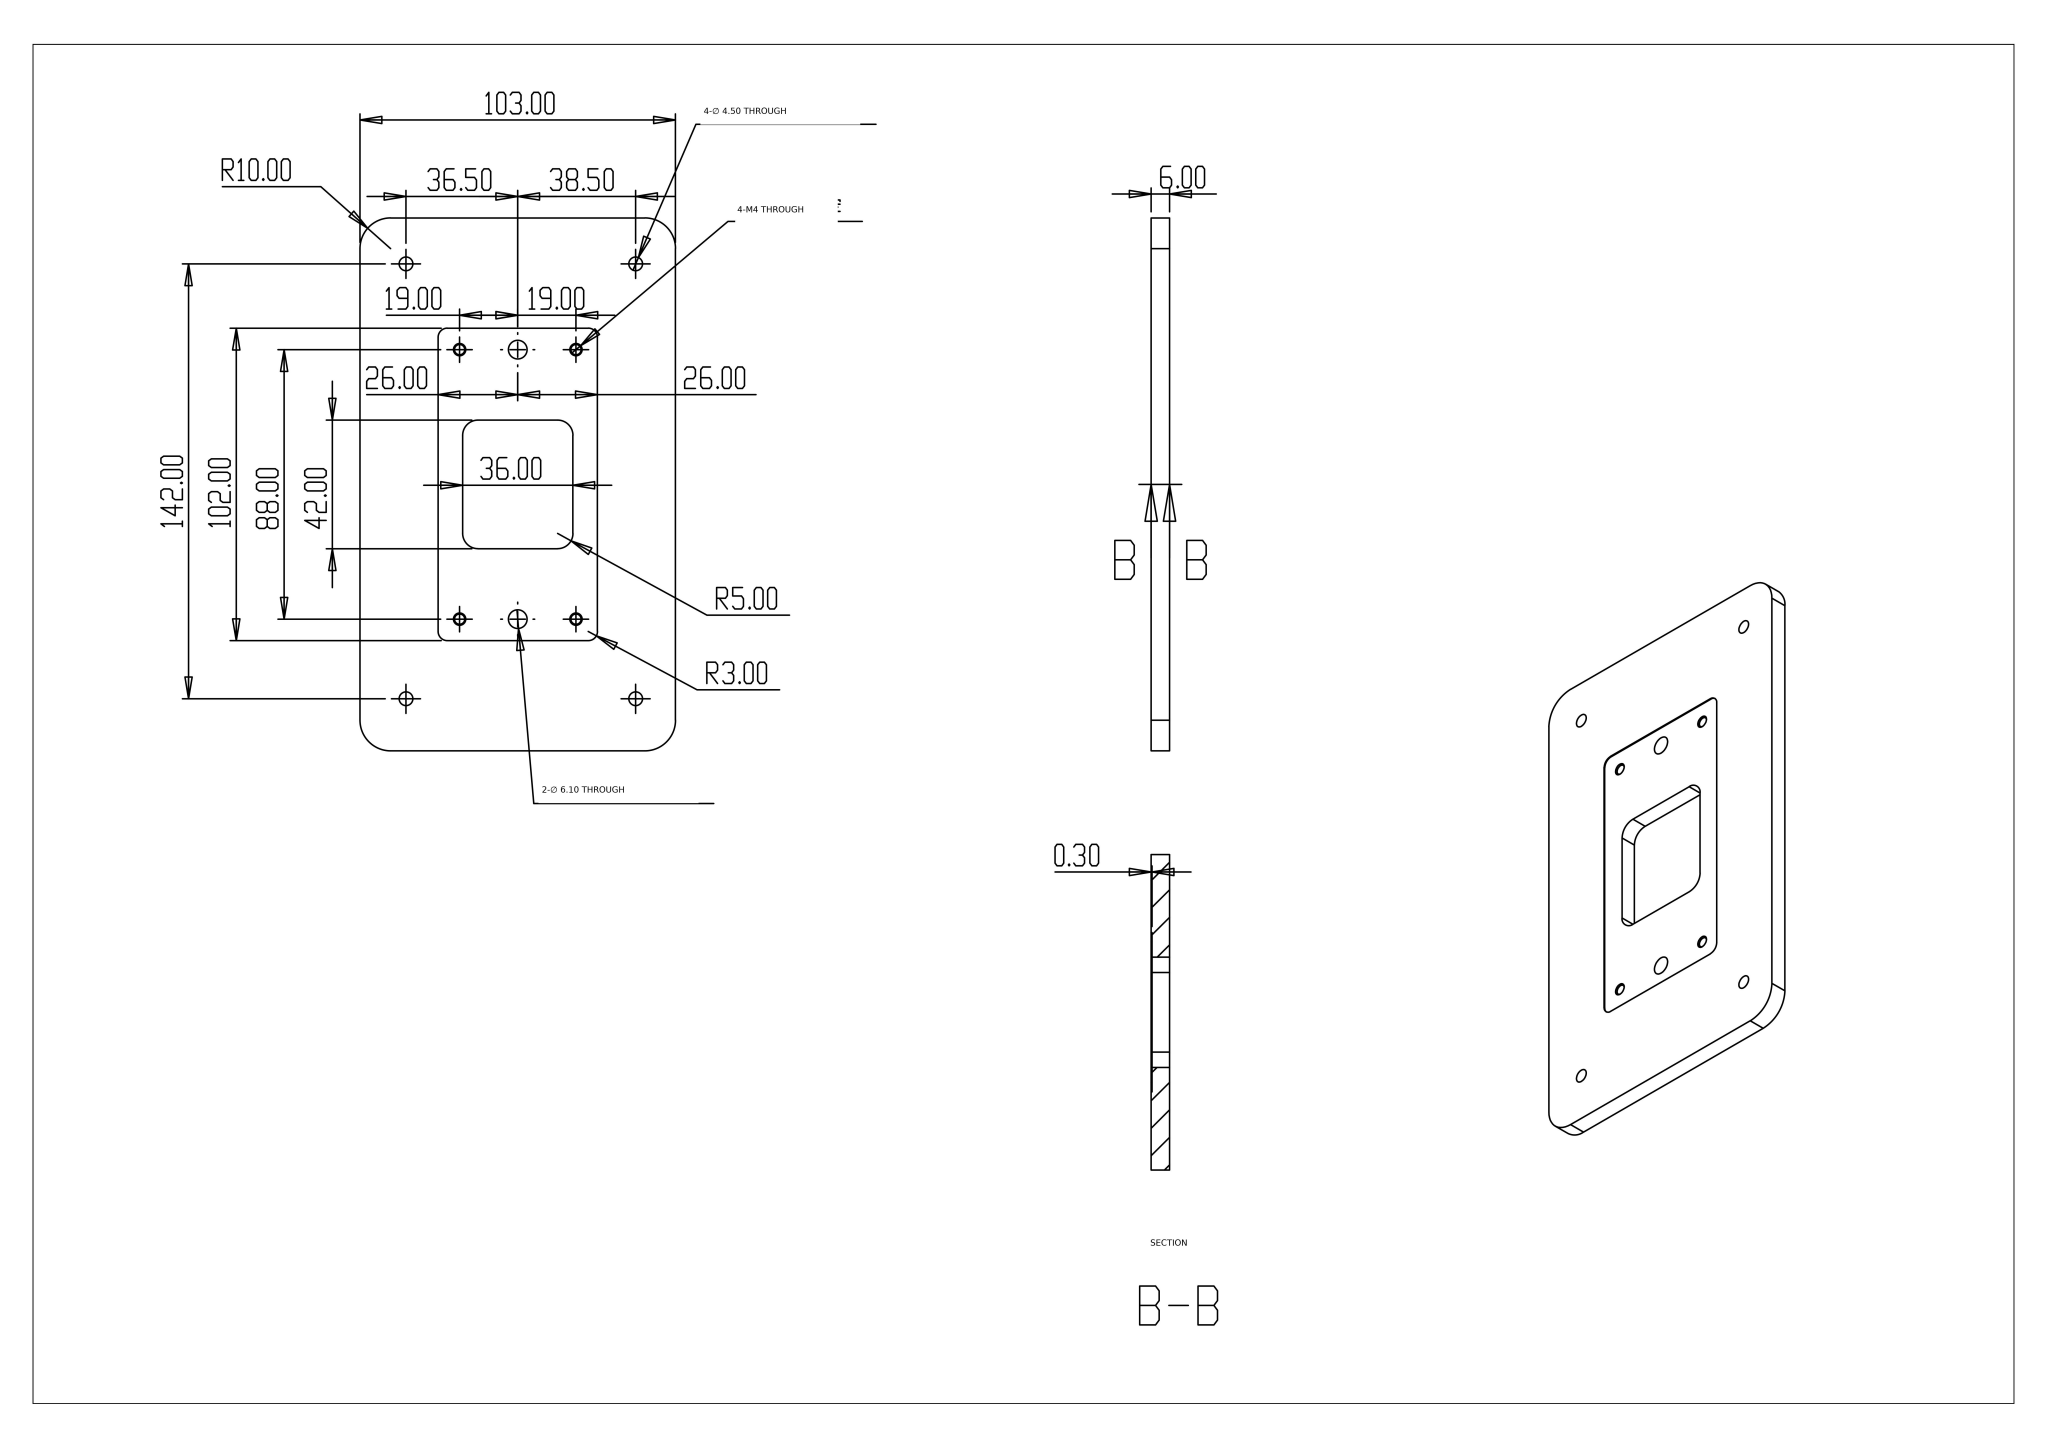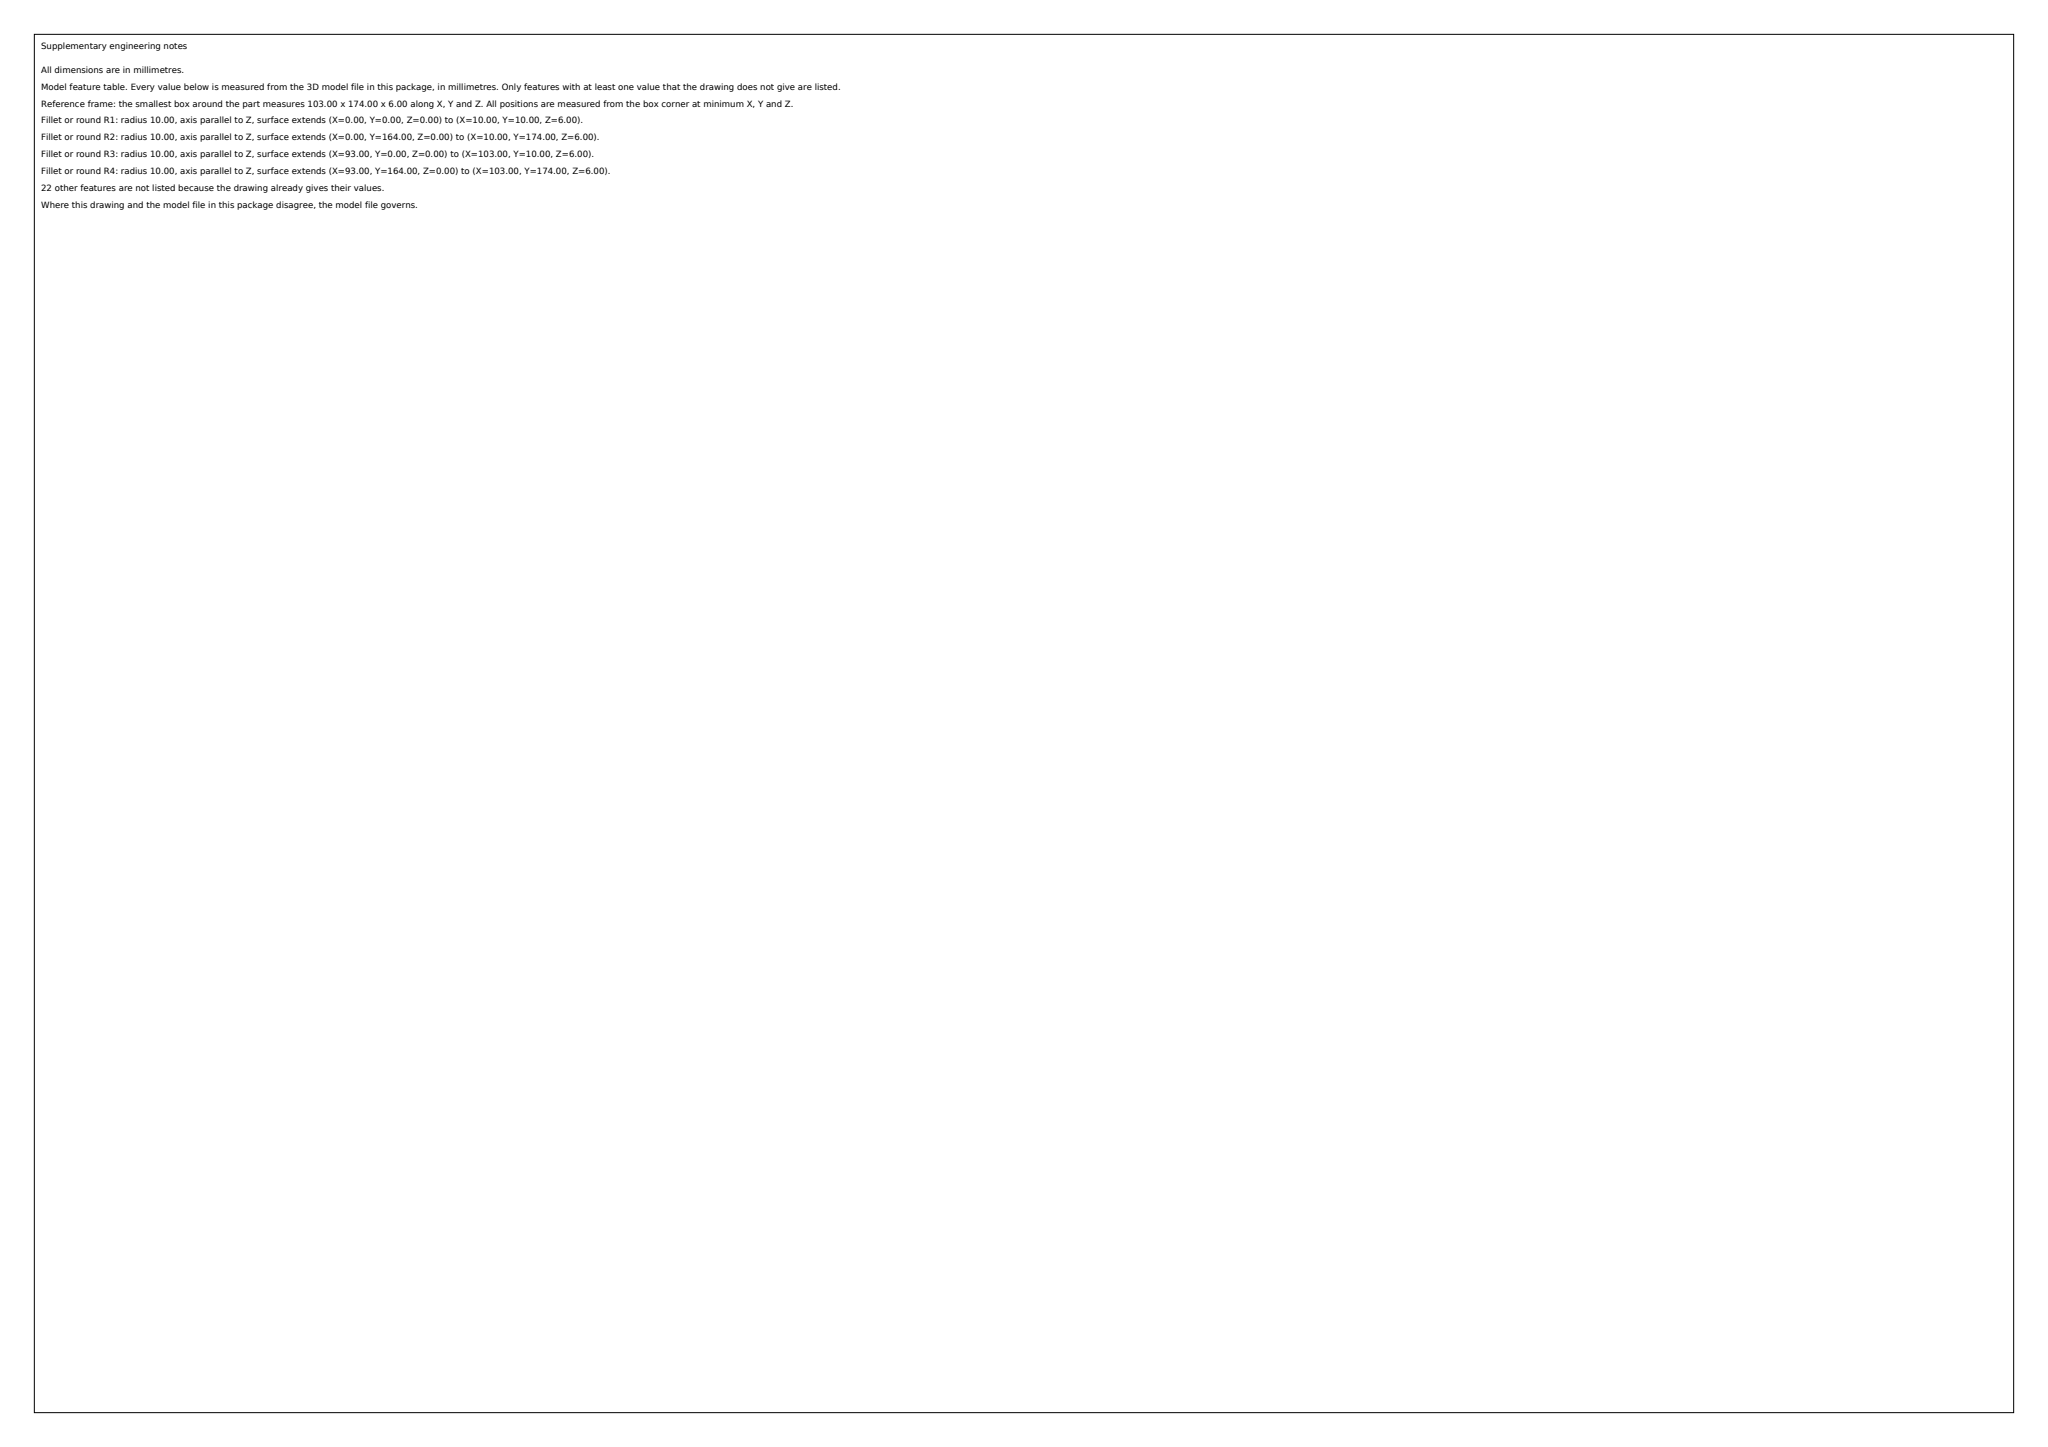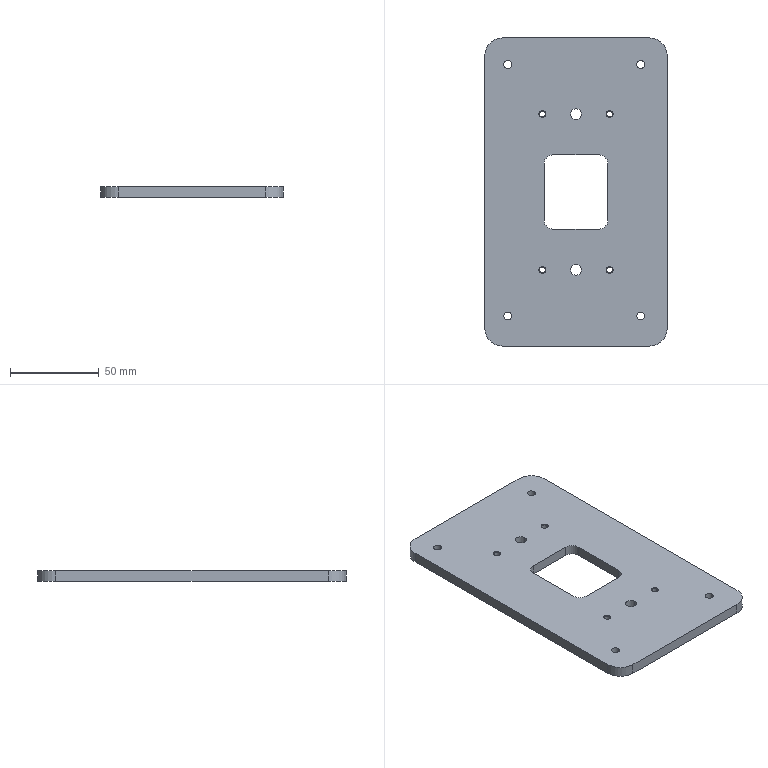Part | SolidWorks | mm | 1 solid | 63 faces | box 103 x 174 x 6 mm | volume 96017 mm3 | cylinder 32 | cone 16 | plane 15 | commonest cylinder face diameters 4.5 x8 3.3 x8 6.1 x4 10 x4 20 x4 6 x4
build123d program:
from build123d import *

# Parameters (mm, degrees)
SKETCH1_R           = 1.65
BOSS_EXTRUDE1_DEPTH = 6
SKETCH2_R           = 1.65
SKETCH2_R_2         = 3.05
CUT_EXTRUDE1_DEPTH  = 0.3
CHAMFER1_SIZE       = 0.35


with BuildPart() as part:
    # Sketch1 → Boss-Extrude1 (new body)
    with BuildSketch(Plane.XY):
        with BuildLine():
            Line((12.899, -45.82), (12.899, 108.18))
            ThreePointArc((12.899, 108.18), (9.97, 115.251), (2.899, 118.18))
            Line((2.899, 118.18), (-80.101, 118.18))
            ThreePointArc((-80.101, 118.18), (-87.172, 115.251), (-90.101, 108.18))
            Line((-90.101, 108.18), (-90.101, -45.82))
            ThreePointArc((-90.101, -45.82), (-87.172, -52.891), (-80.101, -55.82))
            Line((-80.101, -55.82), (2.899, -55.82))
            ThreePointArc((2.899, -55.82), (9.97, -52.891), (12.899, -45.82))
        make_face()
        with Locations((-19.601, 75.18)):
            Circle(SKETCH1_R, mode=Mode.SUBTRACT)
        with Locations((-57.601, 75.18)):
            Circle(SKETCH1_R, mode=Mode.SUBTRACT)
        with Locations((-19.601, -12.82)):
            Circle(SKETCH1_R, mode=Mode.SUBTRACT)
        with Locations((-57.601, -12.82)):
            Circle(SKETCH1_R, mode=Mode.SUBTRACT)
        with BuildLine():
            Line((-25.601, 52.18), (-51.601, 52.18))
            ThreePointArc((-51.601, 52.18), (-55.137, 50.716), (-56.601, 47.18))
            Line((-56.601, 47.18), (-56.601, 15.18))
            ThreePointArc((-56.601, 15.18), (-55.137, 11.645), (-51.601, 10.18))
            Line((-51.601, 10.18), (-25.601, 10.18))
            ThreePointArc((-25.601, 10.18), (-22.066, 11.645), (-20.601, 15.18))
            Line((-20.601, 15.18), (-20.601, 47.18))
            ThreePointArc((-20.601, 47.18), (-22.066, 50.716), (-25.601, 52.18))
        make_face(mode=Mode.SUBTRACT)
        with BuildLine():
            ThreePointArc((0.1487, 103.18), (-2.101, 105.43), (-4.351, 103.18))
            ThreePointArc((-4.351, 103.18), (-2.101, 100.93), (0.1487, 103.18))
        make_face(mode=Mode.SUBTRACT)
        with BuildLine():
            ThreePointArc((-74.851, 103.18), (-77.101, 105.43), (-79.351, 103.18))
            ThreePointArc((-79.351, 103.18), (-77.101, 100.93), (-74.851, 103.18))
        make_face(mode=Mode.SUBTRACT)
        with BuildLine():
            ThreePointArc((-38.601, -9.77), (-41.651, -12.82), (-38.601, -15.87))
            ThreePointArc((-38.601, -15.87), (-35.551, -12.82), (-38.601, -9.77))
        make_face(mode=Mode.SUBTRACT)
        with BuildLine():
            ThreePointArc((-38.601, 78.23), (-41.651, 75.18), (-38.601, 72.13))
            ThreePointArc((-38.601, 72.13), (-35.551, 75.18), (-38.601, 78.23))
        make_face(mode=Mode.SUBTRACT)
        with BuildLine():
            ThreePointArc((0.1487, -38.82), (-2.101, -36.57), (-4.351, -38.82))
            ThreePointArc((-4.351, -38.82), (-2.101, -41.07), (0.1487, -38.82))
        make_face(mode=Mode.SUBTRACT)
        with BuildLine():
            ThreePointArc((-74.851, -38.82), (-77.101, -36.57), (-79.351, -38.82))
            ThreePointArc((-79.351, -38.82), (-77.101, -41.07), (-74.851, -38.82))
        make_face(mode=Mode.SUBTRACT)
    extrude(amount=BOSS_EXTRUDE1_DEPTH)

    # Sketch2 → Cut-Extrude1 (cut)
    with BuildSketch(Plane(origin=(0, 0, 0), x_dir=(-1, 0, 0), z_dir=(0, 0, -1))):
        with BuildLine():
            Line((61.601, 82.18), (15.601, 82.18))
            ThreePointArc((15.601, 82.18), (13.48, 81.301), (12.601, 79.18))
            Line((12.601, 79.18), (12.601, -16.82))
            ThreePointArc((12.601, -16.82), (13.48, -18.941), (15.601, -19.82))
            Line((15.601, -19.82), (61.601, -19.82))
            ThreePointArc((61.601, -19.82), (63.723, -18.941), (64.601, -16.82))
            Line((64.601, -16.82), (64.601, 79.18))
            ThreePointArc((64.601, 79.18), (63.723, 81.301), (61.601, 82.18))
        make_face()
        with Locations((57.601, 75.18)):
            Circle(SKETCH2_R, mode=Mode.SUBTRACT)
        with Locations((38.601, 75.18)):
            Circle(SKETCH2_R_2, mode=Mode.SUBTRACT)
        with Locations((38.601, -12.82)):
            Circle(SKETCH2_R_2, mode=Mode.SUBTRACT)
        with Locations((57.601, -12.82)):
            Circle(SKETCH2_R, mode=Mode.SUBTRACT)
        with Locations((19.601, -12.82)):
            Circle(SKETCH2_R, mode=Mode.SUBTRACT)
        with Locations((19.601, 75.18)):
            Circle(SKETCH2_R, mode=Mode.SUBTRACT)
        with BuildLine():
            Line((25.601, 52.18), (51.601, 52.18))
            ThreePointArc((51.601, 52.18), (55.137, 50.716), (56.601, 47.18))
            Line((56.601, 47.18), (56.601, 15.18))
            ThreePointArc((56.601, 15.18), (55.137, 11.645), (51.601, 10.18))
            Line((51.601, 10.18), (25.601, 10.18))
            ThreePointArc((25.601, 10.18), (22.066, 11.645), (20.601, 15.18))
            Line((20.601, 15.18), (20.601, 47.18))
            ThreePointArc((20.601, 47.18), (22.066, 50.716), (25.601, 52.18))
        make_face(mode=Mode.SUBTRACT)
    extrude(amount=-CUT_EXTRUDE1_DEPTH, mode=Mode.SUBTRACT)

    # Chamfer1
    chamfer1_edges = [part.edges().sort_by_distance(p)[0] for p in [
        (-21.251, 75.18, 0.3),
        (-21.251, -12.82, 0.3),
        (-59.251, -12.82, 0.3),
        (-59.251, 75.18, 0.3),
        (-21.251, 75.18, 6),
        (-59.251, 75.18, 6),
        (-21.251, -12.82, 6),
        (-59.251, -12.82, 6),
    ]]
    chamfer(chamfer1_edges, length=CHAMFER1_SIZE)


solid = part.part